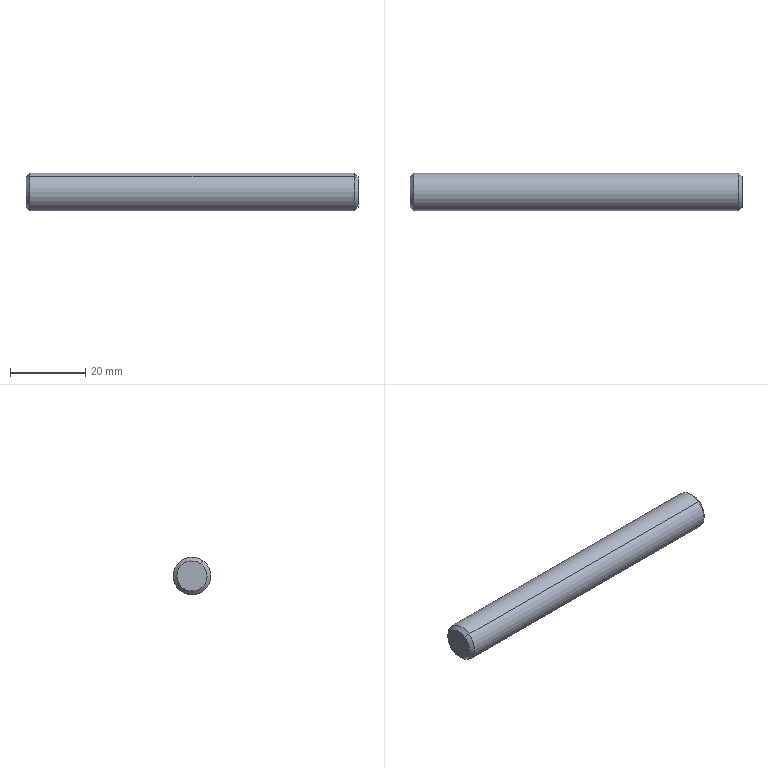Component | SolidWorks | LiftingPlateAssembly-1_LiftingPlateAxis-2 | 1 solid | 8 faces | box 88 x 10 x 10 mm | volume 6882 mm3 | cone 4 | cylinder 2 | plane 2 | commonest cylinder face diameters 10 x2 | material Plain Carbon Steel
build123d program:
from build123d import *

# Parameters (mm, degrees)
SKETCH1_R           = 5
BOSS_EXTRUDE1_DEPTH = 88
CHAMFER1_SIZE       = 1


with BuildPart() as part:
    # Sketch1 → Boss-Extrude1 (new body)
    with BuildSketch(Plane.XY):
        Circle(SKETCH1_R)
    extrude(amount=BOSS_EXTRUDE1_DEPTH)

    # Chamfer1
    chamfer1_edges = [part.edges().sort_by_distance(p)[0] for p in [
        (-5, 0, 0),
        (-5, 0, 88),
    ]]
    chamfer(chamfer1_edges, length=CHAMFER1_SIZE)


solid = part.part

# Placed as in the assembly
solid = solid.moved(Location((-294, 2, -65), (0, 90, 0)))
STEP:
#1=COLOUR_RGB('',0.7922,0.8196,0.9333);
#2=FILL_AREA_STYLE_COLOUR('',#1);
#3=FILL_AREA_STYLE('',(#2));
#4=SURFACE_STYLE_FILL_AREA(#3);
#5=SURFACE_SIDE_STYLE('',(#4));
#6=SURFACE_STYLE_USAGE(.BOTH.,#5);
#7=PRESENTATION_STYLE_ASSIGNMENT((#6));
#8=CARTESIAN_POINT('',(-8.11,-0.01215,-2.43));
#9=VERTEX_POINT('',#8);
#10=CARTESIAN_POINT('',(-8.11,0.1696,-2.688));
#11=VERTEX_POINT('',#10);
#12=CARTESIAN_POINT('',(-8.11,0.07874,-2.559));
#13=DIRECTION('',(1.,0.,-0.));
#14=DIRECTION('',(0.,0.5772,-0.8166));
#15=AXIS2_PLACEMENT_3D('',#12,#13,#14);
#16=CIRCLE('',#15,0.1575);
#17=EDGE_CURVE('',#9,#11,#16,.T.);
#18=ORIENTED_EDGE('',*,*,#17,.F.);
#19=CARTESIAN_POINT('',(-8.15,-0.03488,-2.398));
#20=VERTEX_POINT('',#19);
#21=CARTESIAN_POINT('',(-8.15,-0.03488,-2.398));
#22=DIRECTION('',(-0.7071,-0.4081,0.5774));
#23=VECTOR('',#22,39.37);
#24=LINE('',#21,#23);
#25=EDGE_CURVE('',#9,#20,#24,.T.);
#26=ORIENTED_EDGE('',*,*,#25,.T.);
#27=CARTESIAN_POINT('',(-8.15,0.1924,-2.72));
#28=VERTEX_POINT('',#27);
#29=CARTESIAN_POINT('',(-8.15,0.07874,-2.559));
#30=DIRECTION('',(-1.,-0.,0.));
#31=DIRECTION('',(0.,0.5772,-0.8166));
#32=AXIS2_PLACEMENT_3D('',#29,#30,#31);
#33=CIRCLE('',#32,0.1969);
#34=EDGE_CURVE('',#28,#20,#33,.T.);
#35=ORIENTED_EDGE('',*,*,#34,.F.);
#36=CARTESIAN_POINT('',(-8.15,0.1924,-2.72));
#37=DIRECTION('',(-0.7071,0.4081,-0.5774));
#38=VECTOR('',#37,39.37);
#39=LINE('',#36,#38);
#40=EDGE_CURVE('',#11,#28,#39,.T.);
#41=ORIENTED_EDGE('',*,*,#40,.F.);
#42=EDGE_LOOP('',(#18,#26,#35,#41));
#43=FACE_OUTER_BOUND('',#42,.T.);
#44=CARTESIAN_POINT('',(-8.15,0.07874,-2.559));
#45=DIRECTION('',(-1.,-0.,0.));
#46=DIRECTION('',(0.,0.5772,-0.8166));
#47=AXIS2_PLACEMENT_3D('',#44,#45,#46);
#48=CONICAL_SURFACE('',#47,0.1969,0.7854);
#49=ADVANCED_FACE('',(#43),#48,.T.);
#50=CARTESIAN_POINT('',(-11.575,0.1696,-2.688));
#51=VERTEX_POINT('',#50);
#52=CARTESIAN_POINT('',(-11.575,-0.01215,-2.43));
#53=VERTEX_POINT('',#52);
#54=CARTESIAN_POINT('',(-11.575,0.07874,-2.559));
#55=DIRECTION('',(-1.,-0.,0.));
#56=DIRECTION('',(0.,0.5772,-0.8166));
#57=AXIS2_PLACEMENT_3D('',#54,#55,#56);
#58=CIRCLE('',#57,0.1575);
#59=EDGE_CURVE('',#51,#53,#58,.T.);
#60=ORIENTED_EDGE('',*,*,#59,.F.);
#61=CARTESIAN_POINT('',(-11.535,0.1924,-2.72));
#62=VERTEX_POINT('',#61);
#63=CARTESIAN_POINT('',(-11.575,0.1696,-2.688));
#64=DIRECTION('',(0.7071,0.4081,-0.5774));
#65=VECTOR('',#64,39.37);
#66=LINE('',#63,#65);
#67=EDGE_CURVE('',#51,#62,#66,.T.);
#68=ORIENTED_EDGE('',*,*,#67,.T.);
#69=CARTESIAN_POINT('',(-11.535,-0.03488,-2.398));
#70=VERTEX_POINT('',#69);
#71=CARTESIAN_POINT('',(-11.535,0.07874,-2.559));
#72=DIRECTION('',(1.,0.,-0.));
#73=DIRECTION('',(0.,0.5772,-0.8166));
#74=AXIS2_PLACEMENT_3D('',#71,#72,#73);
#75=CIRCLE('',#74,0.1969);
#76=EDGE_CURVE('',#70,#62,#75,.T.);
#77=ORIENTED_EDGE('',*,*,#76,.F.);
#78=CARTESIAN_POINT('',(-11.575,-0.01215,-2.43));
#79=DIRECTION('',(0.7071,-0.4081,0.5774));
#80=VECTOR('',#79,39.37);
#81=LINE('',#78,#80);
#82=EDGE_CURVE('',#53,#70,#81,.T.);
#83=ORIENTED_EDGE('',*,*,#82,.F.);
#84=EDGE_LOOP('',(#60,#68,#77,#83));
#85=FACE_OUTER_BOUND('',#84,.T.);
#86=CARTESIAN_POINT('',(-11.575,0.07874,-2.559));
#87=DIRECTION('',(1.,0.,-0.));
#88=DIRECTION('',(0.,-0.5772,0.8166));
#89=AXIS2_PLACEMENT_3D('',#86,#87,#88);
#90=CONICAL_SURFACE('',#89,0.1575,0.7854);
#91=ADVANCED_FACE('',(#85),#90,.T.);
#92=ORIENTED_EDGE('',*,*,#76,.T.);
#93=CARTESIAN_POINT('',(-11.575,0.1924,-2.72));
#94=DIRECTION('',(1.,0.,-0.));
#95=VECTOR('',#94,39.37);
#96=LINE('',#93,#95);
#97=EDGE_CURVE('',#62,#28,#96,.T.);
#98=ORIENTED_EDGE('',*,*,#97,.T.);
#99=ORIENTED_EDGE('',*,*,#34,.T.);
#100=CARTESIAN_POINT('',(-11.575,-0.03488,-2.398));
#101=DIRECTION('',(1.,0.,-0.));
#102=VECTOR('',#101,39.37);
#103=LINE('',#100,#102);
#104=EDGE_CURVE('',#70,#20,#103,.T.);
#105=ORIENTED_EDGE('',*,*,#104,.F.);
#106=EDGE_LOOP('',(#92,#98,#99,#105));
#107=FACE_OUTER_BOUND('',#106,.T.);
#108=CARTESIAN_POINT('',(-11.575,0.07874,-2.559));
#109=DIRECTION('',(1.,0.,-0.));
#110=DIRECTION('',(0.,-0.5772,0.8166));
#111=AXIS2_PLACEMENT_3D('',#108,#109,#110);
#112=CYLINDRICAL_SURFACE('',#111,0.1969);
#113=ADVANCED_FACE('',(#107),#112,.T.);
#114=ORIENTED_EDGE('',*,*,#97,.F.);
#115=CARTESIAN_POINT('',(-11.535,0.07874,-2.559));
#116=DIRECTION('',(1.,0.,-0.));
#117=DIRECTION('',(0.,0.5772,-0.8166));
#118=AXIS2_PLACEMENT_3D('',#115,#116,#117);
#119=CIRCLE('',#118,0.1969);
#120=EDGE_CURVE('',#62,#70,#119,.T.);
#121=ORIENTED_EDGE('',*,*,#120,.T.);
#122=ORIENTED_EDGE('',*,*,#104,.T.);
#123=CARTESIAN_POINT('',(-8.15,0.07874,-2.559));
#124=DIRECTION('',(-1.,-0.,0.));
#125=DIRECTION('',(0.,0.5772,-0.8166));
#126=AXIS2_PLACEMENT_3D('',#123,#124,#125);
#127=CIRCLE('',#126,0.1969);
#128=EDGE_CURVE('',#20,#28,#127,.T.);
#129=ORIENTED_EDGE('',*,*,#128,.T.);
#130=EDGE_LOOP('',(#114,#121,#122,#129));
#131=FACE_OUTER_BOUND('',#130,.T.);
#132=CARTESIAN_POINT('',(-11.575,0.07874,-2.559));
#133=DIRECTION('',(1.,0.,-0.));
#134=DIRECTION('',(0.,-0.5772,0.8166));
#135=AXIS2_PLACEMENT_3D('',#132,#133,#134);
#136=CYLINDRICAL_SURFACE('',#135,0.1969);
#137=ADVANCED_FACE('',(#131),#136,.T.);
#138=CARTESIAN_POINT('',(-11.575,0.07874,-2.559));
#139=DIRECTION('',(-1.,-0.,0.));
#140=DIRECTION('',(0.,0.5772,-0.8166));
#141=AXIS2_PLACEMENT_3D('',#138,#139,#140);
#142=CIRCLE('',#141,0.1575);
#143=EDGE_CURVE('',#53,#51,#142,.T.);
#144=ORIENTED_EDGE('',*,*,#143,.T.);
#145=ORIENTED_EDGE('',*,*,#59,.T.);
#146=EDGE_LOOP('',(#144,#145));
#147=FACE_OUTER_BOUND('',#146,.T.);
#148=CARTESIAN_POINT('',(-11.575,0.07874,-2.559));
#149=DIRECTION('',(-1.,-0.,0.));
#150=DIRECTION('',(-0.,0.5772,-0.8166));
#151=AXIS2_PLACEMENT_3D('',#148,#149,#150);
#152=PLANE('',#151);
#153=ADVANCED_FACE('',(#147),#152,.T.);
#154=CARTESIAN_POINT('',(-8.11,0.07874,-2.559));
#155=DIRECTION('',(1.,0.,-0.));
#156=DIRECTION('',(0.,0.5772,-0.8166));
#157=AXIS2_PLACEMENT_3D('',#154,#155,#156);
#158=CIRCLE('',#157,0.1575);
#159=EDGE_CURVE('',#11,#9,#158,.T.);
#160=ORIENTED_EDGE('',*,*,#159,.T.);
#161=ORIENTED_EDGE('',*,*,#17,.T.);
#162=EDGE_LOOP('',(#160,#161));
#163=FACE_OUTER_BOUND('',#162,.T.);
#164=CARTESIAN_POINT('',(-8.11,0.07874,-2.559));
#165=DIRECTION('',(-1.,-0.,0.));
#166=DIRECTION('',(-0.,0.5772,-0.8166));
#167=AXIS2_PLACEMENT_3D('',#164,#165,#166);
#168=PLANE('',#167);
#169=ADVANCED_FACE('',(#163),#168,.F.);
#170=ORIENTED_EDGE('',*,*,#67,.F.);
#171=ORIENTED_EDGE('',*,*,#143,.F.);
#172=ORIENTED_EDGE('',*,*,#82,.T.);
#173=ORIENTED_EDGE('',*,*,#120,.F.);
#174=EDGE_LOOP('',(#170,#171,#172,#173));
#175=FACE_OUTER_BOUND('',#174,.T.);
#176=CARTESIAN_POINT('',(-11.575,0.07874,-2.559));
#177=DIRECTION('',(1.,0.,-0.));
#178=DIRECTION('',(0.,-0.5772,0.8166));
#179=AXIS2_PLACEMENT_3D('',#176,#177,#178);
#180=CONICAL_SURFACE('',#179,0.1575,0.7854);
#181=ADVANCED_FACE('',(#175),#180,.T.);
#182=ORIENTED_EDGE('',*,*,#25,.F.);
#183=ORIENTED_EDGE('',*,*,#159,.F.);
#184=ORIENTED_EDGE('',*,*,#40,.T.);
#185=ORIENTED_EDGE('',*,*,#128,.F.);
#186=EDGE_LOOP('',(#182,#183,#184,#185));
#187=FACE_OUTER_BOUND('',#186,.T.);
#188=CARTESIAN_POINT('',(-8.15,0.07874,-2.559));
#189=DIRECTION('',(-1.,-0.,0.));
#190=DIRECTION('',(0.,0.5772,-0.8166));
#191=AXIS2_PLACEMENT_3D('',#188,#189,#190);
#192=CONICAL_SURFACE('',#191,0.1969,0.7854);
#193=ADVANCED_FACE('',(#187),#192,.T.);
#194=CLOSED_SHELL('',(#49,#91,#113,#137,#153,#169,#181,#193));
#195=MANIFOLD_SOLID_BREP('',#194);
#196=STYLED_ITEM('',(#7),#195);
#197=PRESENTATION_LAYER_ASSIGNMENT('','',(#196));
#198=(LENGTH_UNIT()NAMED_UNIT(*)SI_UNIT($,.METRE.));
#199=LENGTH_MEASURE_WITH_UNIT(LENGTH_MEASURE(0.0254),#198);
#200=DIMENSIONAL_EXPONENTS(1.,0.,0.,0.,0.,0.,0.);
#201=(CONVERSION_BASED_UNIT('',#199)LENGTH_UNIT()NAMED_UNIT(#200));
#202=UNCERTAINTY_MEASURE_WITH_UNIT(LENGTH_MEASURE(0.00001),#201,'','');
#203=(NAMED_UNIT(*)PLANE_ANGLE_UNIT()SI_UNIT($,.RADIAN.));
#204=(NAMED_UNIT(*)SI_UNIT($,.STERADIAN.)SOLID_ANGLE_UNIT());
#205=(GEOMETRIC_REPRESENTATION_CONTEXT(3)GLOBAL_UNCERTAINTY_ASSIGNED_CONTEXT((#202))GLOBAL_UNIT_ASSIGNED_CONTEXT((#201,#203,#204))REPRESENTATION_CONTEXT('',''));
#206=MECHANICAL_DESIGN_GEOMETRIC_PRESENTATION_REPRESENTATION('',(#196),#205);
#207=CARTESIAN_POINT('',(0.,0.,0.));
#208=DIRECTION('',(0.,0.,1.));
#209=DIRECTION('',(1.,0.,0.));
#210=AXIS2_PLACEMENT_3D('',#207,#208,#209);
#211=(LENGTH_UNIT()NAMED_UNIT(*)SI_UNIT($,.METRE.));
#212=LENGTH_MEASURE_WITH_UNIT(LENGTH_MEASURE(0.0254),#211);
#213=DIMENSIONAL_EXPONENTS(1.,0.,0.,0.,0.,0.,0.);
#214=(CONVERSION_BASED_UNIT('',#212)LENGTH_UNIT()NAMED_UNIT(#213));
#215=UNCERTAINTY_MEASURE_WITH_UNIT(LENGTH_MEASURE(0.00001),#214,'','');
#216=(NAMED_UNIT(*)PLANE_ANGLE_UNIT()SI_UNIT($,.RADIAN.));
#217=(NAMED_UNIT(*)SI_UNIT($,.STERADIAN.)SOLID_ANGLE_UNIT());
#218=(GEOMETRIC_REPRESENTATION_CONTEXT(3)GLOBAL_UNCERTAINTY_ASSIGNED_CONTEXT((#215))GLOBAL_UNIT_ASSIGNED_CONTEXT((#214,#216,#217))REPRESENTATION_CONTEXT('',''));
#219=ADVANCED_BREP_SHAPE_REPRESENTATION('',(#195,#210),#218);